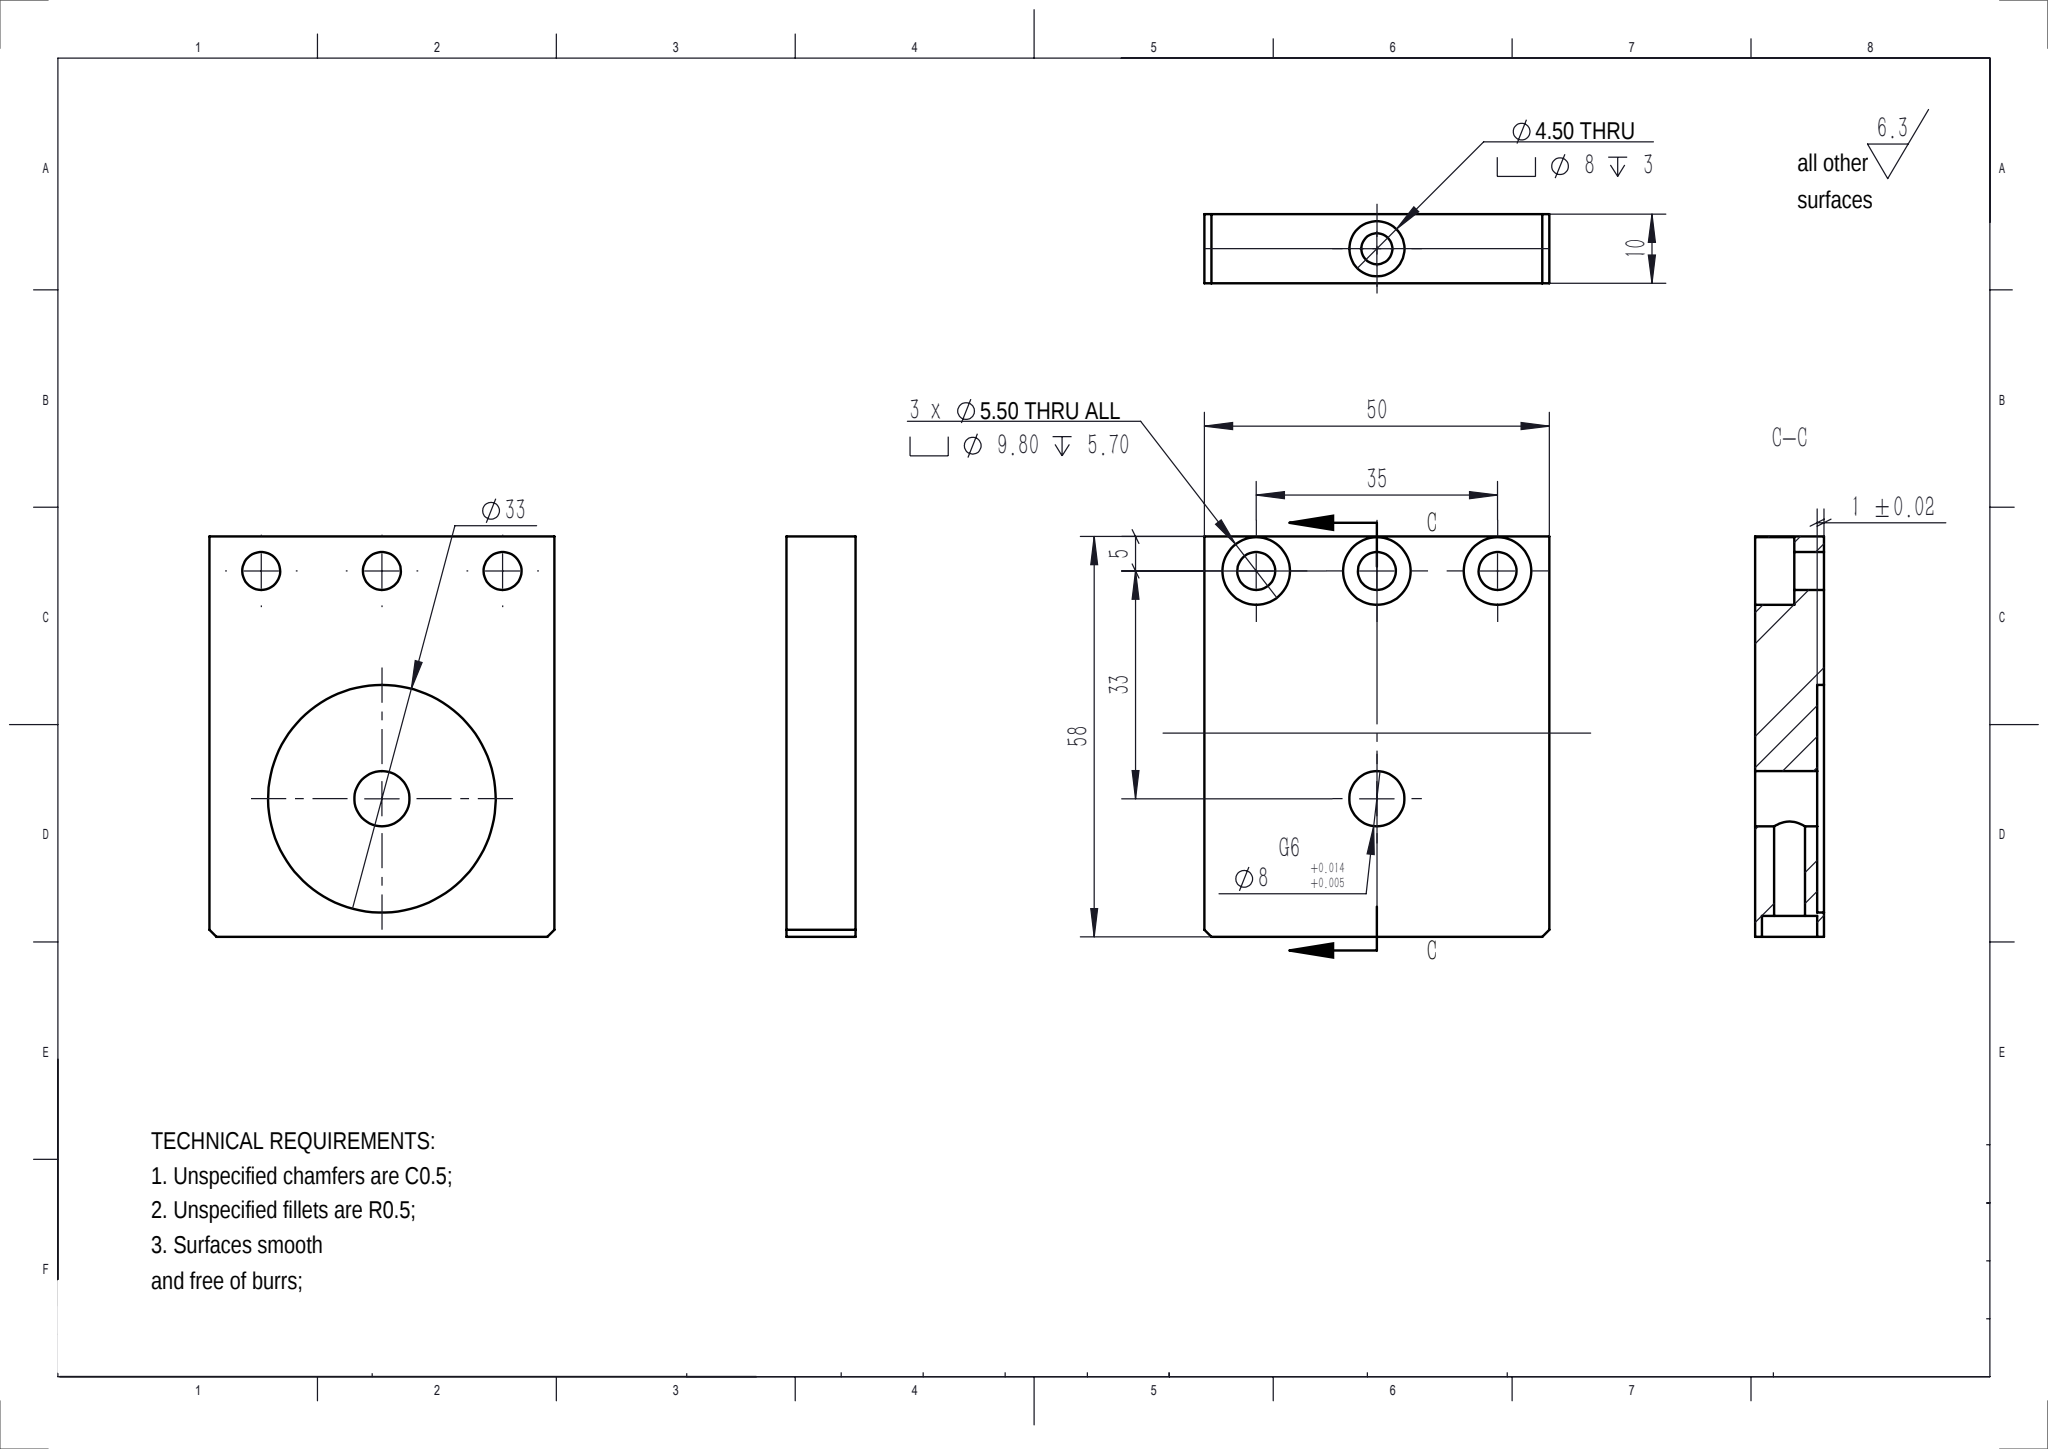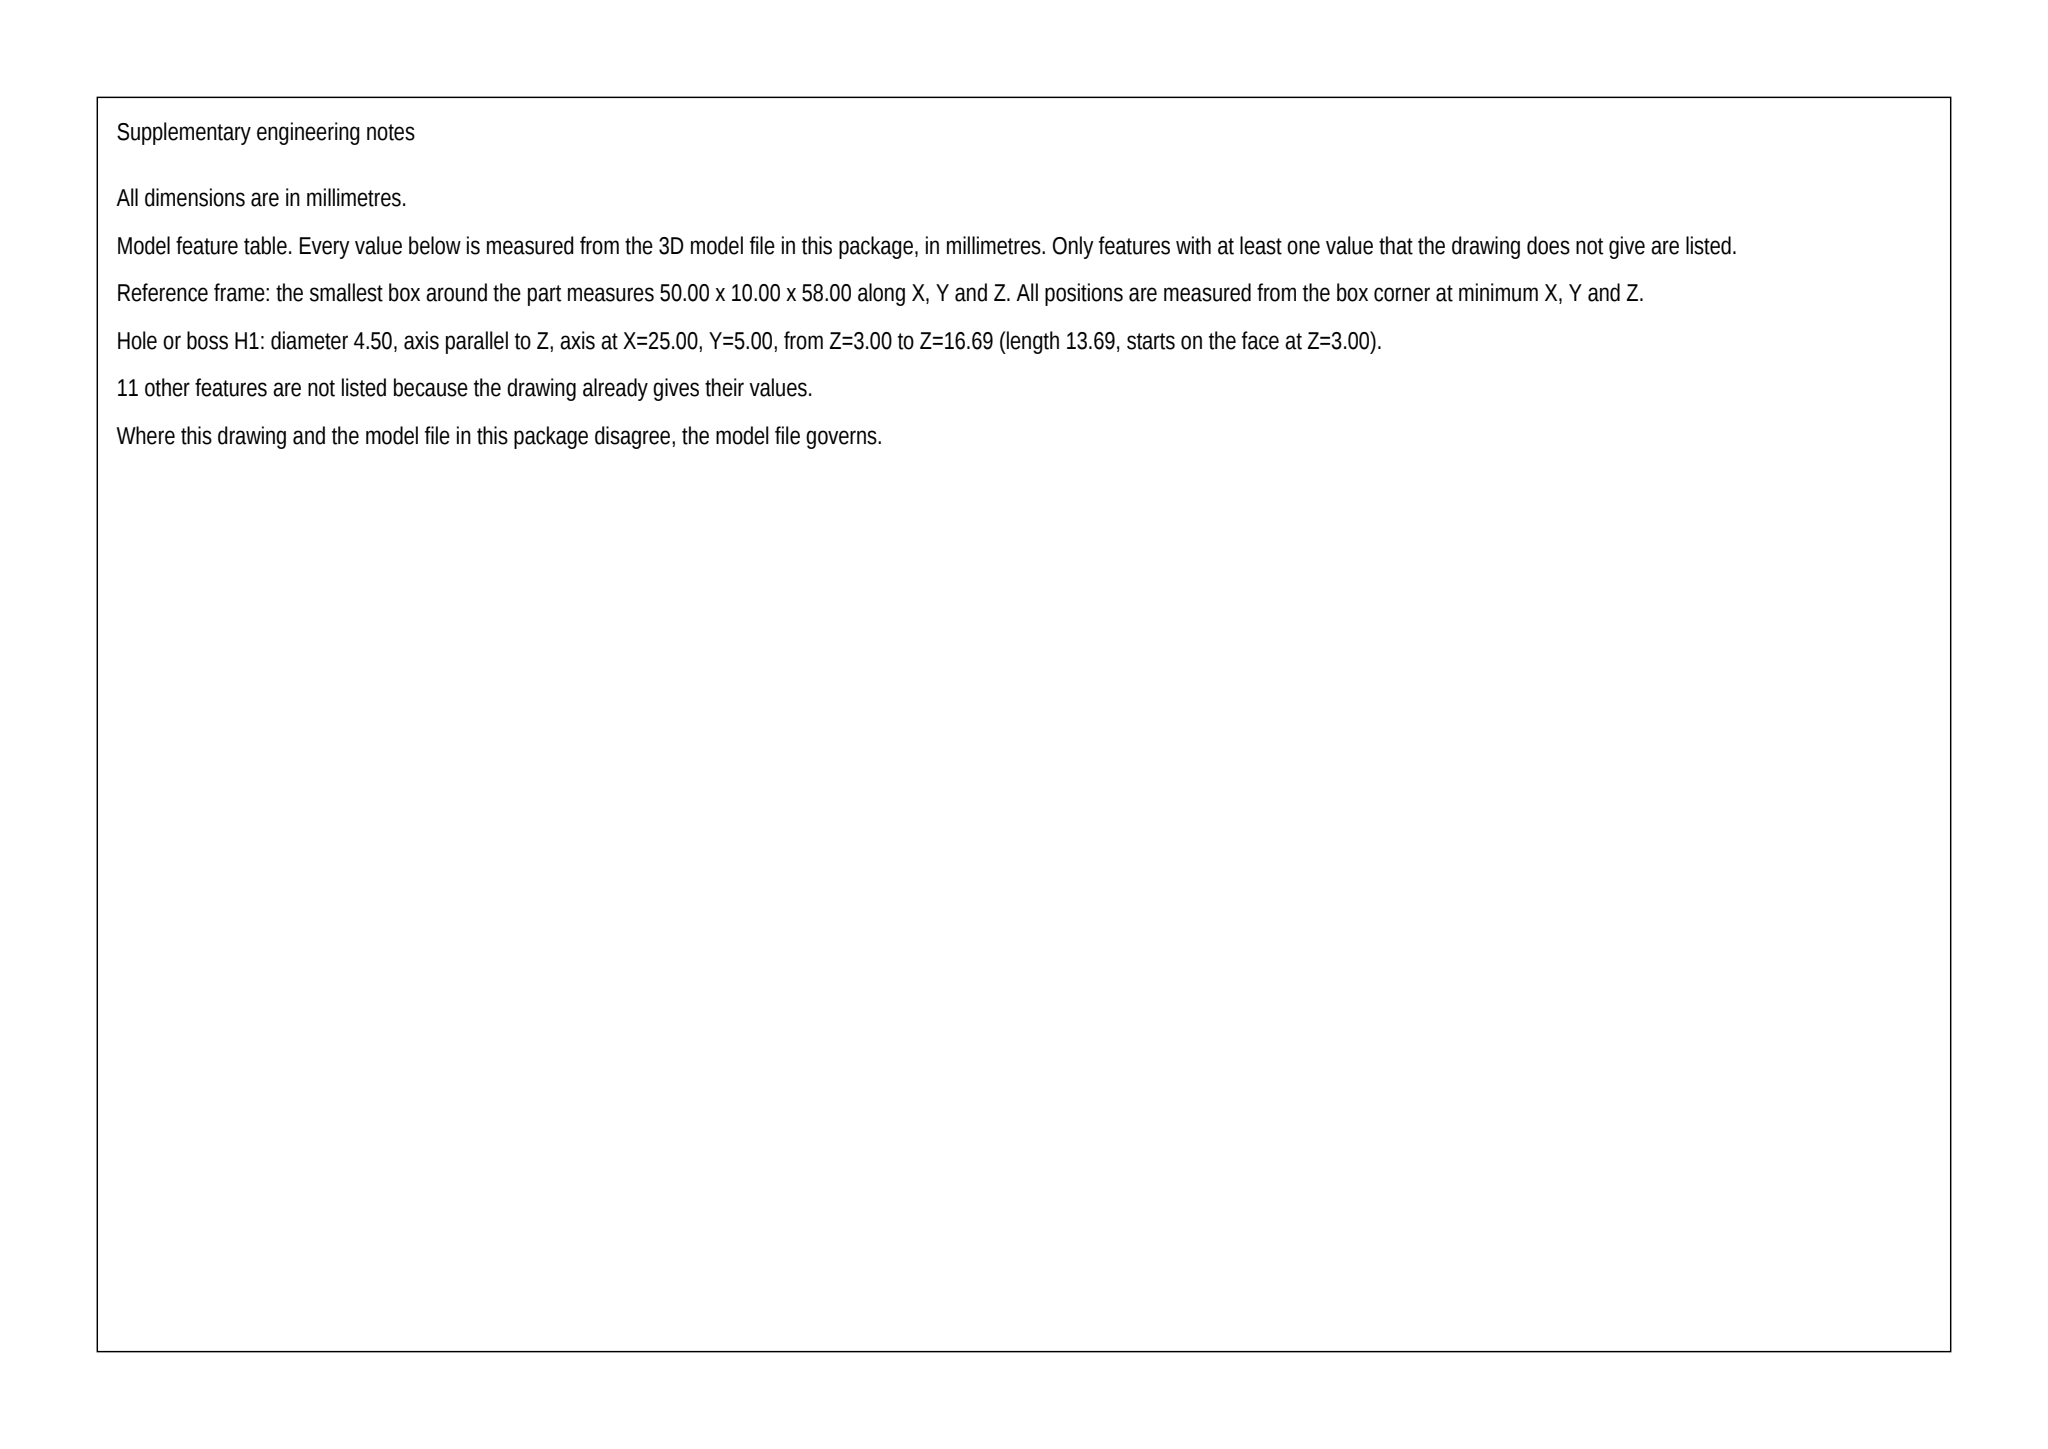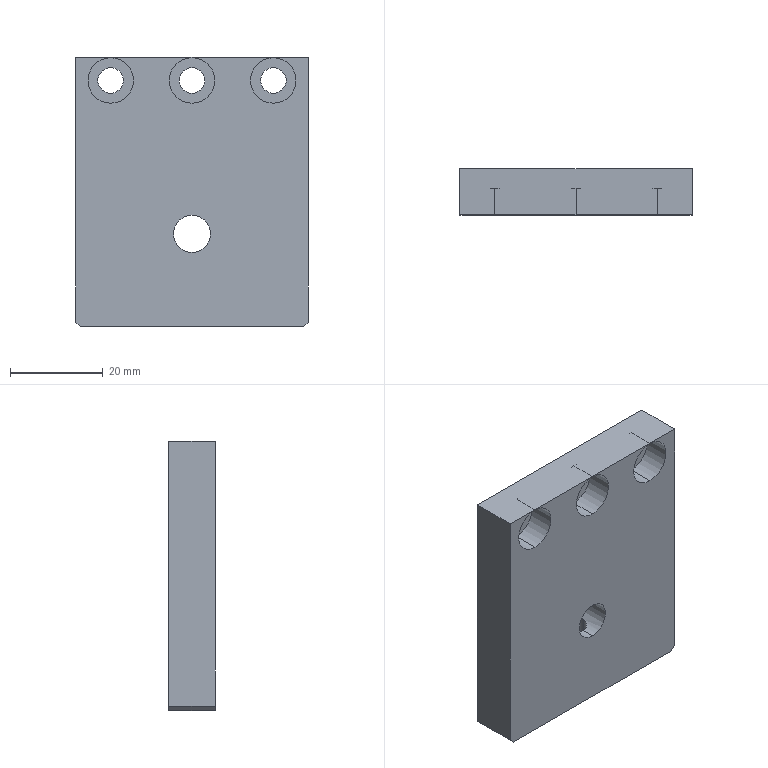Part | SolidWorks | mm | 1 solid | 33 faces | box 50 x 10 x 58 mm | volume 25726 mm3 | cylinder 20 | plane 13 | commonest cylinder face diameters 9.8 x6 5.5 x6 8 x4 4.5 x2 33 x2